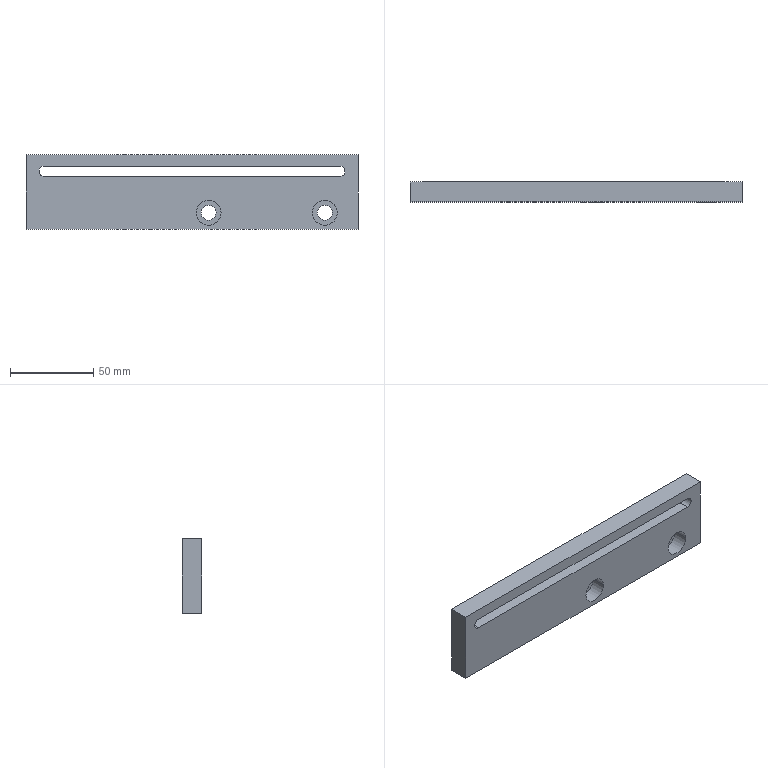Component | SolidWorks | SL021-102-4097.SL4PRT-1 | 1 solid | 21 faces | box 200 x 12 x 45 mm | volume 90607 mm3 | cylinder 11 | plane 10 | commonest cylinder face diameters 15 x4 9 x4 6.3 x3 | material AL6061
build123d program:
from build123d import *

# Parameters (mm, degrees)
SKETCH1_W                                          = 200
SKETCH1_H                                          = 45
BOSS_EXTRUDE1_DEPTH                                = 6
HOLE_SIZE_ACCORDING_TO_TYPE_1_OF_HEXAG_D           = 9
HOLE_SIZE_ACCORDING_TO_TYPE_1_OF_HEXAG_CBORE_D     = 15
HOLE_SIZE_ACCORDING_TO_TYPE_1_OF_HEXAG_CBORE_DEPTH = 9
CUT_EXTRUDE1_DEPTH                                 = 104.2


with BuildPart() as part:
    # Sketch1 → Boss-Extrude1 (new, symmetric)
    with BuildSketch(Plane.XY):
        Rectangle(SKETCH1_W, SKETCH1_H)
    extrude(amount=BOSS_EXTRUDE1_DEPTH, both=True)

    # Hole Size _According to_ Type 1 of Hexag (through all)
    with Locations(Plane(origin=(0, 0, -6), x_dir=(-1, 0, 0), z_dir=(0, 0, -1))):
        with Locations((-10, 12.5), (-80, 12.5)):
            CounterBoreHole(HOLE_SIZE_ACCORDING_TO_TYPE_1_OF_HEXAG_D / 2, HOLE_SIZE_ACCORDING_TO_TYPE_1_OF_HEXAG_CBORE_D / 2, HOLE_SIZE_ACCORDING_TO_TYPE_1_OF_HEXAG_CBORE_DEPTH)

    # Sketch4 → Cut-Extrude1 (cut, through all)
    with BuildSketch(Plane(origin=(0, 0, -6), x_dir=(-1, 0, 0), z_dir=(0, 0, -1))):
        with BuildLine():
            Line((-89, -9.35), (89, -9.35))
            ThreePointArc((89, -9.35), (92.15, -12.5), (89, -15.65))
            Line((89, -15.65), (-89, -15.65))
            ThreePointArc((-89, -15.65), (-92.15, -12.5), (-89, -9.35))
        make_face()
    extrude(amount=-CUT_EXTRUDE1_DEPTH, mode=Mode.SUBTRACT)


solid = part.part

# Placed as in the assembly
solid = solid.moved(Location((-136.163, -96.499, 16.122), (-90, 0, 0)))
STEP:
#1=CARTESIAN_POINT('',(-8.989,-3.563,1.127));
#2=VERTEX_POINT('',#1);
#3=CARTESIAN_POINT('',(-8.865,-3.563,1.003));
#4=VERTEX_POINT('',#3);
#5=CARTESIAN_POINT('',(-8.865,-3.563,1.127));
#6=DIRECTION('',(0.,-1.,0.));
#7=DIRECTION('',(-1.,0.,0.));
#8=AXIS2_PLACEMENT_3D('',#5,#6,#7);
#9=CIRCLE('',#8,0.124);
#10=EDGE_CURVE('',#2,#4,#9,.T.);
#11=ORIENTED_EDGE('',*,*,#10,.F.);
#12=CARTESIAN_POINT('',(-8.989,-4.035,1.127));
#13=VERTEX_POINT('',#12);
#14=CARTESIAN_POINT('',(-8.989,-3.563,1.127));
#15=DIRECTION('',(0.,-1.,0.));
#16=VECTOR('',#15,39.37);
#17=LINE('',#14,#16);
#18=EDGE_CURVE('',#2,#13,#17,.T.);
#19=ORIENTED_EDGE('',*,*,#18,.T.);
#20=CARTESIAN_POINT('',(-8.865,-4.035,1.003));
#21=VERTEX_POINT('',#20);
#22=CARTESIAN_POINT('',(-8.865,-4.035,1.127));
#23=DIRECTION('',(0.,-1.,0.));
#24=DIRECTION('',(-1.,0.,0.));
#25=AXIS2_PLACEMENT_3D('',#22,#23,#24);
#26=CIRCLE('',#25,0.124);
#27=EDGE_CURVE('',#13,#21,#26,.T.);
#28=ORIENTED_EDGE('',*,*,#27,.T.);
#29=CARTESIAN_POINT('',(-8.865,-3.563,1.003));
#30=DIRECTION('',(0.,-1.,0.));
#31=VECTOR('',#30,39.37);
#32=LINE('',#29,#31);
#33=EDGE_CURVE('',#4,#21,#32,.T.);
#34=ORIENTED_EDGE('',*,*,#33,.F.);
#35=EDGE_LOOP('',(#11,#19,#28,#34));
#36=FACE_OUTER_BOUND('',#35,.T.);
#37=CARTESIAN_POINT('',(-8.865,-3.563,1.127));
#38=DIRECTION('',(0.,-1.,0.));
#39=DIRECTION('',(-1.,0.,0.));
#40=AXIS2_PLACEMENT_3D('',#37,#38,#39);
#41=CYLINDRICAL_SURFACE('',#40,0.124);
#42=ADVANCED_FACE('',(#36),#41,.F.);
#43=CARTESIAN_POINT('',(-4.672,-3.681,0.1426));
#44=VERTEX_POINT('',#43);
#45=CARTESIAN_POINT('',(-5.262,-3.681,0.1426));
#46=VERTEX_POINT('',#45);
#47=CARTESIAN_POINT('',(-4.967,-3.681,0.1426));
#48=DIRECTION('',(0.,-1.,0.));
#49=DIRECTION('',(-1.,0.,-0.));
#50=AXIS2_PLACEMENT_3D('',#47,#48,#49);
#51=CIRCLE('',#50,0.2953);
#52=EDGE_CURVE('',#44,#46,#51,.T.);
#53=ORIENTED_EDGE('',*,*,#52,.F.);
#54=CARTESIAN_POINT('',(-4.672,-4.035,0.1426));
#55=VERTEX_POINT('',#54);
#56=CARTESIAN_POINT('',(-4.672,-4.035,0.1426));
#57=DIRECTION('',(0.,-1.,0.));
#58=VECTOR('',#57,39.37);
#59=LINE('',#56,#58);
#60=EDGE_CURVE('',#44,#55,#59,.T.);
#61=ORIENTED_EDGE('',*,*,#60,.T.);
#62=CARTESIAN_POINT('',(-5.262,-4.035,0.1426));
#63=VERTEX_POINT('',#62);
#64=CARTESIAN_POINT('',(-4.967,-4.035,0.1426));
#65=DIRECTION('',(0.,-1.,0.));
#66=DIRECTION('',(-1.,0.,-0.));
#67=AXIS2_PLACEMENT_3D('',#64,#65,#66);
#68=CIRCLE('',#67,0.2953);
#69=EDGE_CURVE('',#55,#63,#68,.T.);
#70=ORIENTED_EDGE('',*,*,#69,.T.);
#71=CARTESIAN_POINT('',(-5.262,-4.035,0.1426));
#72=DIRECTION('',(0.,-1.,0.));
#73=VECTOR('',#72,39.37);
#74=LINE('',#71,#73);
#75=EDGE_CURVE('',#46,#63,#74,.T.);
#76=ORIENTED_EDGE('',*,*,#75,.F.);
#77=EDGE_LOOP('',(#53,#61,#70,#76));
#78=FACE_OUTER_BOUND('',#77,.T.);
#79=CARTESIAN_POINT('',(-4.967,-4.035,0.1426));
#80=DIRECTION('',(0.,-1.,0.));
#81=DIRECTION('',(-1.,0.,-0.));
#82=AXIS2_PLACEMENT_3D('',#79,#80,#81);
#83=CYLINDRICAL_SURFACE('',#82,0.2953);
#84=ADVANCED_FACE('',(#78),#83,.F.);
#85=CARTESIAN_POINT('',(-4.79,-3.563,0.1426));
#86=VERTEX_POINT('',#85);
#87=CARTESIAN_POINT('',(-5.144,-3.563,0.1426));
#88=VERTEX_POINT('',#87);
#89=CARTESIAN_POINT('',(-4.967,-3.563,0.1426));
#90=DIRECTION('',(0.,-1.,0.));
#91=DIRECTION('',(-1.,0.,-0.));
#92=AXIS2_PLACEMENT_3D('',#89,#90,#91);
#93=CIRCLE('',#92,0.1772);
#94=EDGE_CURVE('',#86,#88,#93,.T.);
#95=ORIENTED_EDGE('',*,*,#94,.F.);
#96=CARTESIAN_POINT('',(-4.79,-3.681,0.1426));
#97=VERTEX_POINT('',#96);
#98=CARTESIAN_POINT('',(-4.79,-4.035,0.1426));
#99=DIRECTION('',(0.,-1.,0.));
#100=VECTOR('',#99,39.37);
#101=LINE('',#98,#100);
#102=EDGE_CURVE('',#86,#97,#101,.T.);
#103=ORIENTED_EDGE('',*,*,#102,.T.);
#104=CARTESIAN_POINT('',(-5.144,-3.681,0.1426));
#105=VERTEX_POINT('',#104);
#106=CARTESIAN_POINT('',(-4.967,-3.681,0.1426));
#107=DIRECTION('',(0.,-1.,0.));
#108=DIRECTION('',(-1.,0.,-0.));
#109=AXIS2_PLACEMENT_3D('',#106,#107,#108);
#110=CIRCLE('',#109,0.1772);
#111=EDGE_CURVE('',#97,#105,#110,.T.);
#112=ORIENTED_EDGE('',*,*,#111,.T.);
#113=CARTESIAN_POINT('',(-5.144,-4.035,0.1426));
#114=DIRECTION('',(0.,-1.,0.));
#115=VECTOR('',#114,39.37);
#116=LINE('',#113,#115);
#117=EDGE_CURVE('',#88,#105,#116,.T.);
#118=ORIENTED_EDGE('',*,*,#117,.F.);
#119=EDGE_LOOP('',(#95,#103,#112,#118));
#120=FACE_OUTER_BOUND('',#119,.T.);
#121=CARTESIAN_POINT('',(-4.967,-4.035,0.1426));
#122=DIRECTION('',(0.,-1.,0.));
#123=DIRECTION('',(-1.,0.,-0.));
#124=AXIS2_PLACEMENT_3D('',#121,#122,#123);
#125=CYLINDRICAL_SURFACE('',#124,0.1772);
#126=ADVANCED_FACE('',(#120),#125,.F.);
#127=CARTESIAN_POINT('',(-1.916,-3.681,0.1426));
#128=VERTEX_POINT('',#127);
#129=CARTESIAN_POINT('',(-2.506,-3.681,0.1426));
#130=VERTEX_POINT('',#129);
#131=CARTESIAN_POINT('',(-2.211,-3.681,0.1426));
#132=DIRECTION('',(0.,-1.,0.));
#133=DIRECTION('',(-1.,0.,-0.));
#134=AXIS2_PLACEMENT_3D('',#131,#132,#133);
#135=CIRCLE('',#134,0.2953);
#136=EDGE_CURVE('',#128,#130,#135,.T.);
#137=ORIENTED_EDGE('',*,*,#136,.F.);
#138=CARTESIAN_POINT('',(-1.916,-4.035,0.1426));
#139=VERTEX_POINT('',#138);
#140=CARTESIAN_POINT('',(-1.916,-4.035,0.1426));
#141=DIRECTION('',(0.,-1.,0.));
#142=VECTOR('',#141,39.37);
#143=LINE('',#140,#142);
#144=EDGE_CURVE('',#128,#139,#143,.T.);
#145=ORIENTED_EDGE('',*,*,#144,.T.);
#146=CARTESIAN_POINT('',(-2.506,-4.035,0.1426));
#147=VERTEX_POINT('',#146);
#148=CARTESIAN_POINT('',(-2.211,-4.035,0.1426));
#149=DIRECTION('',(0.,-1.,0.));
#150=DIRECTION('',(-1.,0.,-0.));
#151=AXIS2_PLACEMENT_3D('',#148,#149,#150);
#152=CIRCLE('',#151,0.2953);
#153=EDGE_CURVE('',#139,#147,#152,.T.);
#154=ORIENTED_EDGE('',*,*,#153,.T.);
#155=CARTESIAN_POINT('',(-2.506,-4.035,0.1426));
#156=DIRECTION('',(0.,-1.,0.));
#157=VECTOR('',#156,39.37);
#158=LINE('',#155,#157);
#159=EDGE_CURVE('',#130,#147,#158,.T.);
#160=ORIENTED_EDGE('',*,*,#159,.F.);
#161=EDGE_LOOP('',(#137,#145,#154,#160));
#162=FACE_OUTER_BOUND('',#161,.T.);
#163=CARTESIAN_POINT('',(-2.211,-4.035,0.1426));
#164=DIRECTION('',(0.,-1.,0.));
#165=DIRECTION('',(-1.,0.,-0.));
#166=AXIS2_PLACEMENT_3D('',#163,#164,#165);
#167=CYLINDRICAL_SURFACE('',#166,0.2953);
#168=ADVANCED_FACE('',(#162),#167,.F.);
#169=CARTESIAN_POINT('',(-2.034,-3.563,0.1426));
#170=VERTEX_POINT('',#169);
#171=CARTESIAN_POINT('',(-2.388,-3.563,0.1426));
#172=VERTEX_POINT('',#171);
#173=CARTESIAN_POINT('',(-2.211,-3.563,0.1426));
#174=DIRECTION('',(0.,-1.,0.));
#175=DIRECTION('',(-1.,0.,-0.));
#176=AXIS2_PLACEMENT_3D('',#173,#174,#175);
#177=CIRCLE('',#176,0.1772);
#178=EDGE_CURVE('',#170,#172,#177,.T.);
#179=ORIENTED_EDGE('',*,*,#178,.F.);
#180=CARTESIAN_POINT('',(-2.034,-3.681,0.1426));
#181=VERTEX_POINT('',#180);
#182=CARTESIAN_POINT('',(-2.034,-4.035,0.1426));
#183=DIRECTION('',(0.,-1.,0.));
#184=VECTOR('',#183,39.37);
#185=LINE('',#182,#184);
#186=EDGE_CURVE('',#170,#181,#185,.T.);
#187=ORIENTED_EDGE('',*,*,#186,.T.);
#188=CARTESIAN_POINT('',(-2.388,-3.681,0.1426));
#189=VERTEX_POINT('',#188);
#190=CARTESIAN_POINT('',(-2.211,-3.681,0.1426));
#191=DIRECTION('',(0.,-1.,0.));
#192=DIRECTION('',(-1.,0.,-0.));
#193=AXIS2_PLACEMENT_3D('',#190,#191,#192);
#194=CIRCLE('',#193,0.1772);
#195=EDGE_CURVE('',#181,#189,#194,.T.);
#196=ORIENTED_EDGE('',*,*,#195,.T.);
#197=CARTESIAN_POINT('',(-2.388,-4.035,0.1426));
#198=DIRECTION('',(0.,-1.,0.));
#199=VECTOR('',#198,39.37);
#200=LINE('',#197,#199);
#201=EDGE_CURVE('',#172,#189,#200,.T.);
#202=ORIENTED_EDGE('',*,*,#201,.F.);
#203=EDGE_LOOP('',(#179,#187,#196,#202));
#204=FACE_OUTER_BOUND('',#203,.T.);
#205=CARTESIAN_POINT('',(-2.211,-4.035,0.1426));
#206=DIRECTION('',(0.,-1.,0.));
#207=DIRECTION('',(-1.,0.,-0.));
#208=AXIS2_PLACEMENT_3D('',#205,#206,#207);
#209=CYLINDRICAL_SURFACE('',#208,0.1772);
#210=ADVANCED_FACE('',(#204),#209,.F.);
#211=CARTESIAN_POINT('',(-1.424,-4.035,1.521));
#212=VERTEX_POINT('',#211);
#213=CARTESIAN_POINT('',(-1.424,-4.035,-0.2511));
#214=VERTEX_POINT('',#213);
#215=CARTESIAN_POINT('',(-1.424,-4.035,1.521));
#216=DIRECTION('',(0.,-0.,-1.));
#217=VECTOR('',#216,39.37);
#218=LINE('',#215,#217);
#219=EDGE_CURVE('',#212,#214,#218,.T.);
#220=ORIENTED_EDGE('',*,*,#219,.T.);
#221=CARTESIAN_POINT('',(-1.424,-3.563,-0.2511));
#222=VERTEX_POINT('',#221);
#223=CARTESIAN_POINT('',(-1.424,-3.563,-0.2511));
#224=DIRECTION('',(0.,-1.,0.));
#225=VECTOR('',#224,39.37);
#226=LINE('',#223,#225);
#227=EDGE_CURVE('',#222,#214,#226,.T.);
#228=ORIENTED_EDGE('',*,*,#227,.F.);
#229=CARTESIAN_POINT('',(-1.424,-3.563,1.521));
#230=VERTEX_POINT('',#229);
#231=CARTESIAN_POINT('',(-1.424,-3.563,1.521));
#232=DIRECTION('',(0.,-0.,-1.));
#233=VECTOR('',#232,39.37);
#234=LINE('',#231,#233);
#235=EDGE_CURVE('',#230,#222,#234,.T.);
#236=ORIENTED_EDGE('',*,*,#235,.F.);
#237=CARTESIAN_POINT('',(-1.424,-3.563,1.521));
#238=DIRECTION('',(0.,-1.,0.));
#239=VECTOR('',#238,39.37);
#240=LINE('',#237,#239);
#241=EDGE_CURVE('',#230,#212,#240,.T.);
#242=ORIENTED_EDGE('',*,*,#241,.T.);
#243=EDGE_LOOP('',(#220,#228,#236,#242));
#244=FACE_OUTER_BOUND('',#243,.T.);
#245=CARTESIAN_POINT('',(-1.424,-3.563,1.521));
#246=DIRECTION('',(-1.,-0.,-0.));
#247=DIRECTION('',(-0.,1.,-0.));
#248=AXIS2_PLACEMENT_3D('',#245,#246,#247);
#249=PLANE('',#248);
#250=ADVANCED_FACE('',(#244),#249,.F.);
#251=CARTESIAN_POINT('',(-9.298,-4.035,-0.2511));
#252=VERTEX_POINT('',#251);
#253=CARTESIAN_POINT('',(-9.298,-4.035,-0.2511));
#254=DIRECTION('',(-1.,-0.,-0.));
#255=VECTOR('',#254,39.37);
#256=LINE('',#253,#255);
#257=EDGE_CURVE('',#214,#252,#256,.T.);
#258=ORIENTED_EDGE('',*,*,#257,.T.);
#259=CARTESIAN_POINT('',(-9.298,-3.563,-0.2511));
#260=VERTEX_POINT('',#259);
#261=CARTESIAN_POINT('',(-9.298,-3.563,-0.2511));
#262=DIRECTION('',(0.,-1.,0.));
#263=VECTOR('',#262,39.37);
#264=LINE('',#261,#263);
#265=EDGE_CURVE('',#260,#252,#264,.T.);
#266=ORIENTED_EDGE('',*,*,#265,.F.);
#267=CARTESIAN_POINT('',(-9.298,-3.563,-0.2511));
#268=DIRECTION('',(-1.,-0.,-0.));
#269=VECTOR('',#268,39.37);
#270=LINE('',#267,#269);
#271=EDGE_CURVE('',#222,#260,#270,.T.);
#272=ORIENTED_EDGE('',*,*,#271,.F.);
#273=ORIENTED_EDGE('',*,*,#227,.T.);
#274=EDGE_LOOP('',(#258,#266,#272,#273));
#275=FACE_OUTER_BOUND('',#274,.T.);
#276=CARTESIAN_POINT('',(-9.298,-3.563,-0.2511));
#277=DIRECTION('',(-0.,0.,1.));
#278=DIRECTION('',(0.,-1.,0.));
#279=AXIS2_PLACEMENT_3D('',#276,#277,#278);
#280=PLANE('',#279);
#281=ADVANCED_FACE('',(#275),#280,.F.);
#282=CARTESIAN_POINT('',(-9.298,-4.035,1.521));
#283=VERTEX_POINT('',#282);
#284=CARTESIAN_POINT('',(-9.298,-4.035,1.521));
#285=DIRECTION('',(-0.,0.,1.));
#286=VECTOR('',#285,39.37);
#287=LINE('',#284,#286);
#288=EDGE_CURVE('',#252,#283,#287,.T.);
#289=ORIENTED_EDGE('',*,*,#288,.T.);
#290=CARTESIAN_POINT('',(-9.298,-3.563,1.521));
#291=VERTEX_POINT('',#290);
#292=CARTESIAN_POINT('',(-9.298,-3.563,1.521));
#293=DIRECTION('',(0.,-1.,0.));
#294=VECTOR('',#293,39.37);
#295=LINE('',#292,#294);
#296=EDGE_CURVE('',#291,#283,#295,.T.);
#297=ORIENTED_EDGE('',*,*,#296,.F.);
#298=CARTESIAN_POINT('',(-9.298,-3.563,1.521));
#299=DIRECTION('',(-0.,0.,1.));
#300=VECTOR('',#299,39.37);
#301=LINE('',#298,#300);
#302=EDGE_CURVE('',#260,#291,#301,.T.);
#303=ORIENTED_EDGE('',*,*,#302,.F.);
#304=ORIENTED_EDGE('',*,*,#265,.T.);
#305=EDGE_LOOP('',(#289,#297,#303,#304));
#306=FACE_OUTER_BOUND('',#305,.T.);
#307=CARTESIAN_POINT('',(-9.298,-3.563,1.521));
#308=DIRECTION('',(1.,0.,0.));
#309=DIRECTION('',(0.,-1.,0.));
#310=AXIS2_PLACEMENT_3D('',#307,#308,#309);
#311=PLANE('',#310);
#312=ADVANCED_FACE('',(#306),#311,.F.);
#313=CARTESIAN_POINT('',(-9.298,-4.035,1.521));
#314=DIRECTION('',(1.,0.,0.));
#315=VECTOR('',#314,39.37);
#316=LINE('',#313,#315);
#317=EDGE_CURVE('',#283,#212,#316,.T.);
#318=ORIENTED_EDGE('',*,*,#317,.T.);
#319=ORIENTED_EDGE('',*,*,#241,.F.);
#320=CARTESIAN_POINT('',(-9.298,-3.563,1.521));
#321=DIRECTION('',(1.,0.,0.));
#322=VECTOR('',#321,39.37);
#323=LINE('',#320,#322);
#324=EDGE_CURVE('',#291,#230,#323,.T.);
#325=ORIENTED_EDGE('',*,*,#324,.F.);
#326=ORIENTED_EDGE('',*,*,#296,.T.);
#327=EDGE_LOOP('',(#318,#319,#325,#326));
#328=FACE_OUTER_BOUND('',#327,.T.);
#329=CARTESIAN_POINT('',(-9.298,-3.563,1.521));
#330=DIRECTION('',(0.,-0.,-1.));
#331=DIRECTION('',(-0.,1.,-0.));
#332=AXIS2_PLACEMENT_3D('',#329,#330,#331);
#333=PLANE('',#332);
#334=ADVANCED_FACE('',(#328),#333,.F.);
#335=CARTESIAN_POINT('',(-1.857,-3.563,1.003));
#336=VERTEX_POINT('',#335);
#337=CARTESIAN_POINT('',(-1.857,-3.563,1.003));
#338=DIRECTION('',(1.,0.,0.));
#339=VECTOR('',#338,39.37);
#340=LINE('',#337,#339);
#341=EDGE_CURVE('',#4,#336,#340,.T.);
#342=ORIENTED_EDGE('',*,*,#341,.T.);
#343=CARTESIAN_POINT('',(-1.857,-3.563,1.251));
#344=VERTEX_POINT('',#343);
#345=CARTESIAN_POINT('',(-1.857,-3.563,1.127));
#346=DIRECTION('',(0.,-1.,0.));
#347=DIRECTION('',(-1.,0.,0.));
#348=AXIS2_PLACEMENT_3D('',#345,#346,#347);
#349=CIRCLE('',#348,0.124);
#350=EDGE_CURVE('',#336,#344,#349,.T.);
#351=ORIENTED_EDGE('',*,*,#350,.T.);
#352=CARTESIAN_POINT('',(-8.865,-3.563,1.251));
#353=VERTEX_POINT('',#352);
#354=CARTESIAN_POINT('',(-1.857,-3.563,1.251));
#355=DIRECTION('',(-1.,-0.,-0.));
#356=VECTOR('',#355,39.37);
#357=LINE('',#354,#356);
#358=EDGE_CURVE('',#344,#353,#357,.T.);
#359=ORIENTED_EDGE('',*,*,#358,.T.);
#360=CARTESIAN_POINT('',(-8.865,-3.563,1.127));
#361=DIRECTION('',(0.,-1.,0.));
#362=DIRECTION('',(-1.,0.,0.));
#363=AXIS2_PLACEMENT_3D('',#360,#361,#362);
#364=CIRCLE('',#363,0.124);
#365=EDGE_CURVE('',#353,#2,#364,.T.);
#366=ORIENTED_EDGE('',*,*,#365,.T.);
#367=ORIENTED_EDGE('',*,*,#10,.T.);
#368=EDGE_LOOP('',(#342,#351,#359,#366,#367));
#369=FACE_BOUND('',#368,.T.);
#370=CARTESIAN_POINT('',(-4.967,-3.563,0.1426));
#371=DIRECTION('',(0.,-1.,0.));
#372=DIRECTION('',(-1.,0.,-0.));
#373=AXIS2_PLACEMENT_3D('',#370,#371,#372);
#374=CIRCLE('',#373,0.1772);
#375=EDGE_CURVE('',#88,#86,#374,.T.);
#376=ORIENTED_EDGE('',*,*,#375,.T.);
#377=ORIENTED_EDGE('',*,*,#94,.T.);
#378=EDGE_LOOP('',(#376,#377));
#379=FACE_BOUND('',#378,.T.);
#380=CARTESIAN_POINT('',(-2.211,-3.563,0.1426));
#381=DIRECTION('',(0.,-1.,0.));
#382=DIRECTION('',(-1.,0.,-0.));
#383=AXIS2_PLACEMENT_3D('',#380,#381,#382);
#384=CIRCLE('',#383,0.1772);
#385=EDGE_CURVE('',#172,#170,#384,.T.);
#386=ORIENTED_EDGE('',*,*,#385,.T.);
#387=ORIENTED_EDGE('',*,*,#178,.T.);
#388=EDGE_LOOP('',(#386,#387));
#389=FACE_BOUND('',#388,.T.);
#390=ORIENTED_EDGE('',*,*,#235,.T.);
#391=ORIENTED_EDGE('',*,*,#271,.T.);
#392=ORIENTED_EDGE('',*,*,#302,.T.);
#393=ORIENTED_EDGE('',*,*,#324,.T.);
#394=EDGE_LOOP('',(#390,#391,#392,#393));
#395=FACE_OUTER_BOUND('',#394,.T.);
#396=CARTESIAN_POINT('',(-5.361,-3.563,0.6347));
#397=DIRECTION('',(0.,-1.,0.));
#398=DIRECTION('',(-1.,-0.,-0.));
#399=AXIS2_PLACEMENT_3D('',#396,#397,#398);
#400=PLANE('',#399);
#401=ADVANCED_FACE('',(#369,#379,#389,#395),#400,.F.);
#402=CARTESIAN_POINT('',(-1.857,-4.035,1.003));
#403=VERTEX_POINT('',#402);
#404=CARTESIAN_POINT('',(-1.857,-4.035,1.251));
#405=VERTEX_POINT('',#404);
#406=CARTESIAN_POINT('',(-1.857,-4.035,1.127));
#407=DIRECTION('',(0.,-1.,0.));
#408=DIRECTION('',(-1.,0.,0.));
#409=AXIS2_PLACEMENT_3D('',#406,#407,#408);
#410=CIRCLE('',#409,0.124);
#411=EDGE_CURVE('',#403,#405,#410,.T.);
#412=ORIENTED_EDGE('',*,*,#411,.F.);
#413=CARTESIAN_POINT('',(-1.857,-4.035,1.003));
#414=DIRECTION('',(1.,0.,0.));
#415=VECTOR('',#414,39.37);
#416=LINE('',#413,#415);
#417=EDGE_CURVE('',#21,#403,#416,.T.);
#418=ORIENTED_EDGE('',*,*,#417,.F.);
#419=ORIENTED_EDGE('',*,*,#27,.F.);
#420=CARTESIAN_POINT('',(-8.865,-4.035,1.251));
#421=VERTEX_POINT('',#420);
#422=CARTESIAN_POINT('',(-8.865,-4.035,1.127));
#423=DIRECTION('',(0.,-1.,0.));
#424=DIRECTION('',(-1.,0.,0.));
#425=AXIS2_PLACEMENT_3D('',#422,#423,#424);
#426=CIRCLE('',#425,0.124);
#427=EDGE_CURVE('',#421,#13,#426,.T.);
#428=ORIENTED_EDGE('',*,*,#427,.F.);
#429=CARTESIAN_POINT('',(-1.857,-4.035,1.251));
#430=DIRECTION('',(-1.,-0.,-0.));
#431=VECTOR('',#430,39.37);
#432=LINE('',#429,#431);
#433=EDGE_CURVE('',#405,#421,#432,.T.);
#434=ORIENTED_EDGE('',*,*,#433,.F.);
#435=EDGE_LOOP('',(#412,#418,#419,#428,#434));
#436=FACE_BOUND('',#435,.T.);
#437=CARTESIAN_POINT('',(-4.967,-4.035,0.1426));
#438=DIRECTION('',(0.,-1.,0.));
#439=DIRECTION('',(-1.,0.,-0.));
#440=AXIS2_PLACEMENT_3D('',#437,#438,#439);
#441=CIRCLE('',#440,0.2953);
#442=EDGE_CURVE('',#63,#55,#441,.T.);
#443=ORIENTED_EDGE('',*,*,#442,.F.);
#444=ORIENTED_EDGE('',*,*,#69,.F.);
#445=EDGE_LOOP('',(#443,#444));
#446=FACE_BOUND('',#445,.T.);
#447=CARTESIAN_POINT('',(-2.211,-4.035,0.1426));
#448=DIRECTION('',(0.,-1.,0.));
#449=DIRECTION('',(-1.,0.,-0.));
#450=AXIS2_PLACEMENT_3D('',#447,#448,#449);
#451=CIRCLE('',#450,0.2953);
#452=EDGE_CURVE('',#147,#139,#451,.T.);
#453=ORIENTED_EDGE('',*,*,#452,.F.);
#454=ORIENTED_EDGE('',*,*,#153,.F.);
#455=EDGE_LOOP('',(#453,#454));
#456=FACE_BOUND('',#455,.T.);
#457=ORIENTED_EDGE('',*,*,#219,.F.);
#458=ORIENTED_EDGE('',*,*,#317,.F.);
#459=ORIENTED_EDGE('',*,*,#288,.F.);
#460=ORIENTED_EDGE('',*,*,#257,.F.);
#461=EDGE_LOOP('',(#457,#458,#459,#460));
#462=FACE_OUTER_BOUND('',#461,.T.);
#463=CARTESIAN_POINT('',(-5.361,-4.035,0.6347));
#464=DIRECTION('',(0.,-1.,0.));
#465=DIRECTION('',(-1.,-0.,-0.));
#466=AXIS2_PLACEMENT_3D('',#463,#464,#465);
#467=PLANE('',#466);
#468=ADVANCED_FACE('',(#436,#446,#456,#462),#467,.T.);
#469=ORIENTED_EDGE('',*,*,#186,.F.);
#470=ORIENTED_EDGE('',*,*,#385,.F.);
#471=ORIENTED_EDGE('',*,*,#201,.T.);
#472=CARTESIAN_POINT('',(-2.211,-3.681,0.1426));
#473=DIRECTION('',(0.,-1.,0.));
#474=DIRECTION('',(-1.,0.,-0.));
#475=AXIS2_PLACEMENT_3D('',#472,#473,#474);
#476=CIRCLE('',#475,0.1772);
#477=EDGE_CURVE('',#189,#181,#476,.T.);
#478=ORIENTED_EDGE('',*,*,#477,.T.);
#479=EDGE_LOOP('',(#469,#470,#471,#478));
#480=FACE_OUTER_BOUND('',#479,.T.);
#481=CARTESIAN_POINT('',(-2.211,-4.035,0.1426));
#482=DIRECTION('',(0.,-1.,0.));
#483=DIRECTION('',(-1.,0.,-0.));
#484=AXIS2_PLACEMENT_3D('',#481,#482,#483);
#485=CYLINDRICAL_SURFACE('',#484,0.1772);
#486=ADVANCED_FACE('',(#480),#485,.F.);
#487=ORIENTED_EDGE('',*,*,#477,.F.);
#488=ORIENTED_EDGE('',*,*,#195,.F.);
#489=EDGE_LOOP('',(#487,#488));
#490=FACE_BOUND('',#489,.T.);
#491=CARTESIAN_POINT('',(-2.211,-3.681,0.1426));
#492=DIRECTION('',(0.,-1.,0.));
#493=DIRECTION('',(-1.,0.,-0.));
#494=AXIS2_PLACEMENT_3D('',#491,#492,#493);
#495=CIRCLE('',#494,0.2953);
#496=EDGE_CURVE('',#130,#128,#495,.T.);
#497=ORIENTED_EDGE('',*,*,#496,.T.);
#498=ORIENTED_EDGE('',*,*,#136,.T.);
#499=EDGE_LOOP('',(#497,#498));
#500=FACE_OUTER_BOUND('',#499,.T.);
#501=CARTESIAN_POINT('',(-2.034,-3.681,0.1426));
#502=DIRECTION('',(-0.,1.,-0.));
#503=DIRECTION('',(1.,0.,0.));
#504=AXIS2_PLACEMENT_3D('',#501,#502,#503);
#505=PLANE('',#504);
#506=ADVANCED_FACE('',(#490,#500),#505,.F.);
#507=ORIENTED_EDGE('',*,*,#144,.F.);
#508=ORIENTED_EDGE('',*,*,#496,.F.);
#509=ORIENTED_EDGE('',*,*,#159,.T.);
#510=ORIENTED_EDGE('',*,*,#452,.T.);
#511=EDGE_LOOP('',(#507,#508,#509,#510));
#512=FACE_OUTER_BOUND('',#511,.T.);
#513=CARTESIAN_POINT('',(-2.211,-4.035,0.1426));
#514=DIRECTION('',(0.,-1.,0.));
#515=DIRECTION('',(-1.,0.,-0.));
#516=AXIS2_PLACEMENT_3D('',#513,#514,#515);
#517=CYLINDRICAL_SURFACE('',#516,0.2953);
#518=ADVANCED_FACE('',(#512),#517,.F.);
#519=ORIENTED_EDGE('',*,*,#102,.F.);
#520=ORIENTED_EDGE('',*,*,#375,.F.);
#521=ORIENTED_EDGE('',*,*,#117,.T.);
#522=CARTESIAN_POINT('',(-4.967,-3.681,0.1426));
#523=DIRECTION('',(0.,-1.,0.));
#524=DIRECTION('',(-1.,0.,-0.));
#525=AXIS2_PLACEMENT_3D('',#522,#523,#524);
#526=CIRCLE('',#525,0.1772);
#527=EDGE_CURVE('',#105,#97,#526,.T.);
#528=ORIENTED_EDGE('',*,*,#527,.T.);
#529=EDGE_LOOP('',(#519,#520,#521,#528));
#530=FACE_OUTER_BOUND('',#529,.T.);
#531=CARTESIAN_POINT('',(-4.967,-4.035,0.1426));
#532=DIRECTION('',(0.,-1.,0.));
#533=DIRECTION('',(-1.,0.,-0.));
#534=AXIS2_PLACEMENT_3D('',#531,#532,#533);
#535=CYLINDRICAL_SURFACE('',#534,0.1772);
#536=ADVANCED_FACE('',(#530),#535,.F.);
#537=ORIENTED_EDGE('',*,*,#527,.F.);
#538=ORIENTED_EDGE('',*,*,#111,.F.);
#539=EDGE_LOOP('',(#537,#538));
#540=FACE_BOUND('',#539,.T.);
#541=CARTESIAN_POINT('',(-4.967,-3.681,0.1426));
#542=DIRECTION('',(0.,-1.,0.));
#543=DIRECTION('',(-1.,0.,-0.));
#544=AXIS2_PLACEMENT_3D('',#541,#542,#543);
#545=CIRCLE('',#544,0.2953);
#546=EDGE_CURVE('',#46,#44,#545,.T.);
#547=ORIENTED_EDGE('',*,*,#546,.T.);
#548=ORIENTED_EDGE('',*,*,#52,.T.);
#549=EDGE_LOOP('',(#547,#548));
#550=FACE_OUTER_BOUND('',#549,.T.);
#551=CARTESIAN_POINT('',(-4.79,-3.681,0.1426));
#552=DIRECTION('',(-0.,1.,-0.));
#553=DIRECTION('',(1.,0.,0.));
#554=AXIS2_PLACEMENT_3D('',#551,#552,#553);
#555=PLANE('',#554);
#556=ADVANCED_FACE('',(#540,#550),#555,.F.);
#557=ORIENTED_EDGE('',*,*,#60,.F.);
#558=ORIENTED_EDGE('',*,*,#546,.F.);
#559=ORIENTED_EDGE('',*,*,#75,.T.);
#560=ORIENTED_EDGE('',*,*,#442,.T.);
#561=EDGE_LOOP('',(#557,#558,#559,#560));
#562=FACE_OUTER_BOUND('',#561,.T.);
#563=CARTESIAN_POINT('',(-4.967,-4.035,0.1426));
#564=DIRECTION('',(0.,-1.,0.));
#565=DIRECTION('',(-1.,0.,-0.));
#566=AXIS2_PLACEMENT_3D('',#563,#564,#565);
#567=CYLINDRICAL_SURFACE('',#566,0.2953);
#568=ADVANCED_FACE('',(#562),#567,.F.);
#569=ORIENTED_EDGE('',*,*,#411,.T.);
#570=CARTESIAN_POINT('',(-1.857,-3.563,1.251));
#571=DIRECTION('',(0.,-1.,0.));
#572=VECTOR('',#571,39.37);
#573=LINE('',#570,#572);
#574=EDGE_CURVE('',#344,#405,#573,.T.);
#575=ORIENTED_EDGE('',*,*,#574,.F.);
#576=ORIENTED_EDGE('',*,*,#350,.F.);
#577=CARTESIAN_POINT('',(-1.857,-3.563,1.003));
#578=DIRECTION('',(0.,-1.,0.));
#579=VECTOR('',#578,39.37);
#580=LINE('',#577,#579);
#581=EDGE_CURVE('',#336,#403,#580,.T.);
#582=ORIENTED_EDGE('',*,*,#581,.T.);
#583=EDGE_LOOP('',(#569,#575,#576,#582));
#584=FACE_OUTER_BOUND('',#583,.T.);
#585=CARTESIAN_POINT('',(-1.857,-3.563,1.127));
#586=DIRECTION('',(0.,-1.,0.));
#587=DIRECTION('',(-1.,0.,0.));
#588=AXIS2_PLACEMENT_3D('',#585,#586,#587);
#589=CYLINDRICAL_SURFACE('',#588,0.124);
#590=ADVANCED_FACE('',(#584),#589,.F.);
#591=ORIENTED_EDGE('',*,*,#417,.T.);
#592=ORIENTED_EDGE('',*,*,#581,.F.);
#593=ORIENTED_EDGE('',*,*,#341,.F.);
#594=ORIENTED_EDGE('',*,*,#33,.T.);
#595=EDGE_LOOP('',(#591,#592,#593,#594));
#596=FACE_OUTER_BOUND('',#595,.T.);
#597=CARTESIAN_POINT('',(-1.857,-3.563,1.003));
#598=DIRECTION('',(0.,-0.,-1.));
#599=DIRECTION('',(-0.,1.,-0.));
#600=AXIS2_PLACEMENT_3D('',#597,#598,#599);
#601=PLANE('',#600);
#602=ADVANCED_FACE('',(#596),#601,.F.);
#603=ORIENTED_EDGE('',*,*,#18,.F.);
#604=ORIENTED_EDGE('',*,*,#365,.F.);
#605=CARTESIAN_POINT('',(-8.865,-3.563,1.251));
#606=DIRECTION('',(0.,-1.,0.));
#607=VECTOR('',#606,39.37);
#608=LINE('',#605,#607);
#609=EDGE_CURVE('',#353,#421,#608,.T.);
#610=ORIENTED_EDGE('',*,*,#609,.T.);
#611=ORIENTED_EDGE('',*,*,#427,.T.);
#612=EDGE_LOOP('',(#603,#604,#610,#611));
#613=FACE_OUTER_BOUND('',#612,.T.);
#614=CARTESIAN_POINT('',(-8.865,-3.563,1.127));
#615=DIRECTION('',(0.,-1.,0.));
#616=DIRECTION('',(-1.,0.,0.));
#617=AXIS2_PLACEMENT_3D('',#614,#615,#616);
#618=CYLINDRICAL_SURFACE('',#617,0.124);
#619=ADVANCED_FACE('',(#613),#618,.F.);
#620=ORIENTED_EDGE('',*,*,#433,.T.);
#621=ORIENTED_EDGE('',*,*,#609,.F.);
#622=ORIENTED_EDGE('',*,*,#358,.F.);
#623=ORIENTED_EDGE('',*,*,#574,.T.);
#624=EDGE_LOOP('',(#620,#621,#622,#623));
#625=FACE_OUTER_BOUND('',#624,.T.);
#626=CARTESIAN_POINT('',(-1.857,-3.563,1.251));
#627=DIRECTION('',(-0.,0.,1.));
#628=DIRECTION('',(0.,-1.,0.));
#629=AXIS2_PLACEMENT_3D('',#626,#627,#628);
#630=PLANE('',#629);
#631=ADVANCED_FACE('',(#625),#630,.F.);
#632=CLOSED_SHELL('',(#42,#84,#126,#168,#210,#250,#281,#312,#334,#401,#468,#486,#506,#518,#536,#556,#568,#590,#602,#619,#631));
#633=MANIFOLD_SOLID_BREP('',#632);
#634=CARTESIAN_POINT('',(0.,0.,0.));
#635=DIRECTION('',(0.,0.,1.));
#636=DIRECTION('',(1.,0.,0.));
#637=AXIS2_PLACEMENT_3D('',#634,#635,#636);
#638=(LENGTH_UNIT()NAMED_UNIT(*)SI_UNIT($,.METRE.));
#639=LENGTH_MEASURE_WITH_UNIT(LENGTH_MEASURE(0.0254),#638);
#640=DIMENSIONAL_EXPONENTS(1.,0.,0.,0.,0.,0.,0.);
#641=(CONVERSION_BASED_UNIT('',#639)LENGTH_UNIT()NAMED_UNIT(#640));
#642=UNCERTAINTY_MEASURE_WITH_UNIT(LENGTH_MEASURE(0.00001),#641,'','');
#643=(NAMED_UNIT(*)PLANE_ANGLE_UNIT()SI_UNIT($,.RADIAN.));
#644=(NAMED_UNIT(*)SI_UNIT($,.STERADIAN.)SOLID_ANGLE_UNIT());
#645=(GEOMETRIC_REPRESENTATION_CONTEXT(3)GLOBAL_UNCERTAINTY_ASSIGNED_CONTEXT((#642))GLOBAL_UNIT_ASSIGNED_CONTEXT((#641,#643,#644))REPRESENTATION_CONTEXT('',''));
#646=ADVANCED_BREP_SHAPE_REPRESENTATION('',(#633,#637),#645);
#647=COLOUR_RGB('',0.7922,0.8196,0.9333);
#648=FILL_AREA_STYLE_COLOUR('',#647);
#649=FILL_AREA_STYLE('',(#648));
#650=SURFACE_STYLE_FILL_AREA(#649);
#651=SURFACE_SIDE_STYLE('',(#650));
#652=SURFACE_STYLE_USAGE(.BOTH.,#651);
#653=PRESENTATION_STYLE_ASSIGNMENT((#652));
#654=STYLED_ITEM('',(#653),#633);
#655=PRESENTATION_LAYER_ASSIGNMENT('','',(#654));
#656=(LENGTH_UNIT()NAMED_UNIT(*)SI_UNIT($,.METRE.));
#657=LENGTH_MEASURE_WITH_UNIT(LENGTH_MEASURE(0.0254),#656);
#658=DIMENSIONAL_EXPONENTS(1.,0.,0.,0.,0.,0.,0.);
#659=(CONVERSION_BASED_UNIT('',#657)LENGTH_UNIT()NAMED_UNIT(#658));
#660=UNCERTAINTY_MEASURE_WITH_UNIT(LENGTH_MEASURE(0.00001),#659,'','');
#661=(NAMED_UNIT(*)PLANE_ANGLE_UNIT()SI_UNIT($,.RADIAN.));
#662=(NAMED_UNIT(*)SI_UNIT($,.STERADIAN.)SOLID_ANGLE_UNIT());
#663=(GEOMETRIC_REPRESENTATION_CONTEXT(3)GLOBAL_UNCERTAINTY_ASSIGNED_CONTEXT((#660))GLOBAL_UNIT_ASSIGNED_CONTEXT((#659,#661,#662))REPRESENTATION_CONTEXT('',''));
#664=MECHANICAL_DESIGN_GEOMETRIC_PRESENTATION_REPRESENTATION('',(#654),#663);